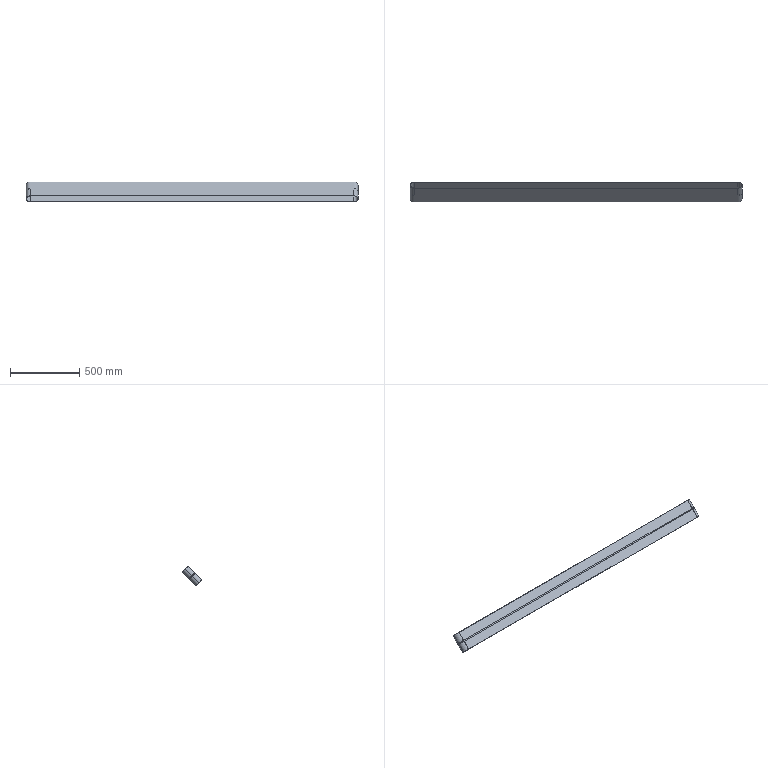Component | SolidWorks | Belt-2 | 1 solid | 32 faces | box 2398 x 143.9 x 143.9 mm | volume 1137609 mm3 | plane 14 | cylinder 12 | cone 6 | commonest cylinder face diameters 60 x6 52 x3 63 x3
build123d program:
from build123d import *

# Parameters (mm, degrees)
EXTRUDE_THIN1_DEPTH = 70


with BuildPart() as part:
    # Sketch1 → Extrude-Thin1 (new, symmetric)
    with BuildSketch(Plane.XY):
        with BuildLine():
            Line((-1167.5, 31.5), (1167.5, 31.5))
            ThreePointArc((1167.5, 31.5), (1199, 0), (1167.5, -31.5))
            Line((1167.5, -31.5), (-1167.5, -31.5))
            ThreePointArc((-1167.5, -31.5), (-1199, 0), (-1167.5, 31.5))
        make_face()
        with BuildLine():
            Line((-1167.5, 30), (1167.5, 30))
            ThreePointArc((1167.5, 30), (1197.5, 0), (1167.5, -30))
            Line((1167.5, -30), (-1167.5, -30))
            ThreePointArc((-1167.5, -30), (-1197.5, 0), (-1167.5, 30))
        make_face(mode=Mode.SUBTRACT)
    extrude(amount=EXTRUDE_THIN1_DEPTH, both=True)

    # Sweep1: sweep along a path in Sketch3
    with BuildLine(Plane.XY) as sweep1_path:
        Line((-1167.5, 30), (1167.5, 30))
        ThreePointArc((1167.5, 30), (1197.5, 0), (1167.5, -30))
        Line((1167.5, -30), (-1167.5, -30))
        ThreePointArc((-1167.5, -30), (-1197.5, 0), (-1167.5, 30))
    # Sketch2 → Sweep1 (sweep)
    with BuildSketch(Plane(origin=(0, 0, 0), x_dir=(0, 0, -1), z_dir=(1, 0, 0))):
        Polygon((-4, -30), (4, -30), (2, -26), (-2, -26), align=None)
    sweep(path=sweep1_path.line)


solid = part.part

# Placed as in the assembly
solid = solid.moved(Location((1065.5, 709.045, 342.308), (-45, 0, -0.01232)))
STEP:
#1=CARTESIAN_POINT('',(-5.039,27.867,13.414));
#2=VERTEX_POINT('',#1);
#3=CARTESIAN_POINT('',(-4.016,28.59,12.69));
#4=VERTEX_POINT('',#3);
#5=CARTESIAN_POINT('',(-4.016,27.866,13.414));
#6=DIRECTION('',(0.,-0.7071,-0.7071));
#7=DIRECTION('',(-1.,0.000152,-0.000152));
#8=AXIS2_PLACEMENT_3D('',#5,#6,#7);
#9=CIRCLE('',#8,1.024);
#10=EDGE_CURVE('',#2,#4,#9,.T.);
#11=ORIENTED_EDGE('',*,*,#10,.F.);
#12=CARTESIAN_POINT('',(-5.197,27.811,13.358));
#13=VERTEX_POINT('',#12);
#14=CARTESIAN_POINT('',(-5.197,27.811,13.358));
#15=DIRECTION('',(-0.8944,-0.3161,-0.3164));
#16=VECTOR('',#15,39.37);
#17=LINE('',#14,#16);
#18=EDGE_CURVE('',#2,#13,#17,.T.);
#19=ORIENTED_EDGE('',*,*,#18,.T.);
#20=CARTESIAN_POINT('',(-4.015,28.646,12.523));
#21=VERTEX_POINT('',#20);
#22=CARTESIAN_POINT('',(-4.016,27.811,13.358));
#23=DIRECTION('',(0.,-0.7071,-0.7071));
#24=DIRECTION('',(-1.,0.000152,-0.000152));
#25=AXIS2_PLACEMENT_3D('',#22,#23,#24);
#26=CIRCLE('',#25,1.181);
#27=EDGE_CURVE('',#13,#21,#26,.T.);
#28=ORIENTED_EDGE('',*,*,#27,.T.);
#29=CARTESIAN_POINT('',(-4.015,28.646,12.523));
#30=DIRECTION('',(-0.0001923,-0.3162,0.9487));
#31=VECTOR('',#30,39.37);
#32=LINE('',#29,#31);
#33=EDGE_CURVE('',#21,#4,#32,.T.);
#34=ORIENTED_EDGE('',*,*,#33,.T.);
#35=EDGE_LOOP('',(#11,#19,#28,#34));
#36=FACE_OUTER_BOUND('',#35,.T.);
#37=CARTESIAN_POINT('',(-4.016,27.811,13.358));
#38=DIRECTION('',(0.,-0.7071,-0.7071));
#39=DIRECTION('',(-1.,0.000152,-0.000152));
#40=AXIS2_PLACEMENT_3D('',#37,#38,#39);
#41=CONICAL_SURFACE('',#40,1.181,1.107);
#42=ADVANCED_FACE('',(#36),#41,.F.);
#43=CARTESIAN_POINT('',(-5.039,27.978,13.525));
#44=VERTEX_POINT('',#43);
#45=CARTESIAN_POINT('',(-4.016,28.702,12.802));
#46=VERTEX_POINT('',#45);
#47=CARTESIAN_POINT('',(-4.016,27.978,13.525));
#48=DIRECTION('',(0.,-0.7071,-0.7071));
#49=DIRECTION('',(-1.,0.000152,-0.000152));
#50=AXIS2_PLACEMENT_3D('',#47,#48,#49);
#51=CIRCLE('',#50,1.024);
#52=EDGE_CURVE('',#44,#46,#51,.T.);
#53=ORIENTED_EDGE('',*,*,#52,.F.);
#54=CARTESIAN_POINT('',(-5.039,27.922,13.47));
#55=DIRECTION('',(0.,-0.7071,-0.7071));
#56=VECTOR('',#55,39.37);
#57=LINE('',#54,#56);
#58=EDGE_CURVE('',#44,#2,#57,.T.);
#59=ORIENTED_EDGE('',*,*,#58,.T.);
#60=ORIENTED_EDGE('',*,*,#10,.T.);
#61=CARTESIAN_POINT('',(-4.016,28.59,12.69));
#62=DIRECTION('',(-0.,0.7071,0.7071));
#63=VECTOR('',#62,39.37);
#64=LINE('',#61,#63);
#65=EDGE_CURVE('',#4,#46,#64,.T.);
#66=ORIENTED_EDGE('',*,*,#65,.T.);
#67=EDGE_LOOP('',(#53,#59,#60,#66));
#68=FACE_OUTER_BOUND('',#67,.T.);
#69=CARTESIAN_POINT('',(-4.016,27.922,13.47));
#70=DIRECTION('',(0.,-0.7071,-0.7071));
#71=DIRECTION('',(-1.,0.000152,-0.000152));
#72=AXIS2_PLACEMENT_3D('',#69,#70,#71);
#73=CYLINDRICAL_SURFACE('',#72,1.024);
#74=ADVANCED_FACE('',(#68),#73,.F.);
#75=CARTESIAN_POINT('',(87.914,28.688,12.816));
#76=VERTEX_POINT('',#75);
#77=CARTESIAN_POINT('',(88.937,27.964,13.54));
#78=VERTEX_POINT('',#77);
#79=CARTESIAN_POINT('',(87.913,27.964,13.539));
#80=DIRECTION('',(0.,-0.7071,-0.7071));
#81=DIRECTION('',(-1.,0.000152,-0.000152));
#82=AXIS2_PLACEMENT_3D('',#79,#80,#81);
#83=CIRCLE('',#82,1.024);
#84=EDGE_CURVE('',#76,#78,#83,.T.);
#85=ORIENTED_EDGE('',*,*,#84,.T.);
#86=CARTESIAN_POINT('',(89.094,28.019,13.595));
#87=VERTEX_POINT('',#86);
#88=CARTESIAN_POINT('',(88.937,27.964,13.54));
#89=DIRECTION('',(0.8944,0.3161,0.3164));
#90=VECTOR('',#89,39.37);
#91=LINE('',#88,#90);
#92=EDGE_CURVE('',#78,#87,#91,.T.);
#93=ORIENTED_EDGE('',*,*,#92,.T.);
#94=CARTESIAN_POINT('',(87.914,28.855,12.76));
#95=VERTEX_POINT('',#94);
#96=CARTESIAN_POINT('',(87.913,28.02,13.595));
#97=DIRECTION('',(0.,-0.7071,-0.7071));
#98=DIRECTION('',(-1.,0.000152,-0.000152));
#99=AXIS2_PLACEMENT_3D('',#96,#97,#98);
#100=CIRCLE('',#99,1.181);
#101=EDGE_CURVE('',#95,#87,#100,.T.);
#102=ORIENTED_EDGE('',*,*,#101,.F.);
#103=CARTESIAN_POINT('',(87.914,28.688,12.816));
#104=DIRECTION('',(0.0001923,0.9487,-0.3162));
#105=VECTOR('',#104,39.37);
#106=LINE('',#103,#105);
#107=EDGE_CURVE('',#76,#95,#106,.T.);
#108=ORIENTED_EDGE('',*,*,#107,.F.);
#109=EDGE_LOOP('',(#85,#93,#102,#108));
#110=FACE_OUTER_BOUND('',#109,.T.);
#111=CARTESIAN_POINT('',(87.913,27.964,13.539));
#112=DIRECTION('',(-0.,0.7071,0.7071));
#113=DIRECTION('',(1.,-0.000152,0.000152));
#114=AXIS2_PLACEMENT_3D('',#111,#112,#113);
#115=CONICAL_SURFACE('',#114,1.024,1.107);
#116=ADVANCED_FACE('',(#110),#115,.F.);
#117=CARTESIAN_POINT('',(-5.256,29.871,15.418));
#118=VERTEX_POINT('',#117);
#119=CARTESIAN_POINT('',(-4.016,28.994,16.295));
#120=VERTEX_POINT('',#119);
#121=CARTESIAN_POINT('',(-4.016,29.871,15.418));
#122=DIRECTION('',(-0.,0.7071,0.7071));
#123=DIRECTION('',(1.,-0.000152,0.000152));
#124=AXIS2_PLACEMENT_3D('',#121,#122,#123);
#125=CIRCLE('',#124,1.24);
#126=EDGE_CURVE('',#118,#120,#125,.T.);
#127=ORIENTED_EDGE('',*,*,#126,.F.);
#128=CARTESIAN_POINT('',(-5.256,25.974,11.521));
#129=VERTEX_POINT('',#128);
#130=CARTESIAN_POINT('',(-5.256,29.871,15.418));
#131=DIRECTION('',(0.,-0.7071,-0.7071));
#132=VECTOR('',#131,39.37);
#133=LINE('',#130,#132);
#134=EDGE_CURVE('',#118,#129,#133,.T.);
#135=ORIENTED_EDGE('',*,*,#134,.T.);
#136=CARTESIAN_POINT('',(-4.016,25.096,12.398));
#137=VERTEX_POINT('',#136);
#138=CARTESIAN_POINT('',(-4.016,25.973,11.521));
#139=DIRECTION('',(-0.,0.7071,0.7071));
#140=DIRECTION('',(1.,-0.000152,0.000152));
#141=AXIS2_PLACEMENT_3D('',#138,#139,#140);
#142=CIRCLE('',#141,1.24);
#143=EDGE_CURVE('',#129,#137,#142,.T.);
#144=ORIENTED_EDGE('',*,*,#143,.T.);
#145=CARTESIAN_POINT('',(-4.016,28.994,16.295));
#146=DIRECTION('',(0.,-0.7071,-0.7071));
#147=VECTOR('',#146,39.37);
#148=LINE('',#145,#147);
#149=EDGE_CURVE('',#120,#137,#148,.T.);
#150=ORIENTED_EDGE('',*,*,#149,.F.);
#151=EDGE_LOOP('',(#127,#135,#144,#150));
#152=FACE_OUTER_BOUND('',#151,.T.);
#153=CARTESIAN_POINT('',(-4.016,29.871,15.418));
#154=DIRECTION('',(0.,-0.7071,-0.7071));
#155=DIRECTION('',(-1.,0.000152,-0.000152));
#156=AXIS2_PLACEMENT_3D('',#153,#154,#155);
#157=CYLINDRICAL_SURFACE('',#156,1.24);
#158=ADVANCED_FACE('',(#152),#157,.T.);
#159=CARTESIAN_POINT('',(-4.015,30.706,14.583));
#160=VERTEX_POINT('',#159);
#161=CARTESIAN_POINT('',(-5.197,29.871,15.418));
#162=VERTEX_POINT('',#161);
#163=CARTESIAN_POINT('',(-4.016,29.871,15.418));
#164=DIRECTION('',(-0.,0.7071,0.7071));
#165=DIRECTION('',(1.,-0.000152,0.000152));
#166=AXIS2_PLACEMENT_3D('',#163,#164,#165);
#167=CIRCLE('',#166,1.181);
#168=EDGE_CURVE('',#160,#162,#167,.T.);
#169=ORIENTED_EDGE('',*,*,#168,.T.);
#170=CARTESIAN_POINT('',(-5.197,28.034,13.581));
#171=VERTEX_POINT('',#170);
#172=CARTESIAN_POINT('',(-5.197,29.871,15.418));
#173=DIRECTION('',(0.,-0.7071,-0.7071));
#174=VECTOR('',#173,39.37);
#175=LINE('',#172,#174);
#176=EDGE_CURVE('',#162,#171,#175,.T.);
#177=ORIENTED_EDGE('',*,*,#176,.T.);
#178=CARTESIAN_POINT('',(-4.015,28.869,12.746));
#179=VERTEX_POINT('',#178);
#180=CARTESIAN_POINT('',(-4.016,28.033,13.581));
#181=DIRECTION('',(0.,-0.7071,-0.7071));
#182=DIRECTION('',(-1.,0.000152,-0.000152));
#183=AXIS2_PLACEMENT_3D('',#180,#181,#182);
#184=CIRCLE('',#183,1.181);
#185=EDGE_CURVE('',#171,#179,#184,.T.);
#186=ORIENTED_EDGE('',*,*,#185,.T.);
#187=CARTESIAN_POINT('',(-4.015,30.706,14.583));
#188=DIRECTION('',(0.,-0.7071,-0.7071));
#189=VECTOR('',#188,39.37);
#190=LINE('',#187,#189);
#191=EDGE_CURVE('',#160,#179,#190,.T.);
#192=ORIENTED_EDGE('',*,*,#191,.F.);
#193=EDGE_LOOP('',(#169,#177,#186,#192));
#194=FACE_OUTER_BOUND('',#193,.T.);
#195=CARTESIAN_POINT('',(-4.016,29.871,15.418));
#196=DIRECTION('',(0.,-0.7071,-0.7071));
#197=DIRECTION('',(-1.,0.000152,-0.000152));
#198=AXIS2_PLACEMENT_3D('',#195,#196,#197);
#199=CYLINDRICAL_SURFACE('',#198,1.181);
#200=ADVANCED_FACE('',(#194),#199,.F.);
#201=ORIENTED_EDGE('',*,*,#27,.F.);
#202=CARTESIAN_POINT('',(-5.197,25.974,11.521));
#203=VERTEX_POINT('',#202);
#204=CARTESIAN_POINT('',(-5.197,29.871,15.418));
#205=DIRECTION('',(0.,-0.7071,-0.7071));
#206=VECTOR('',#205,39.37);
#207=LINE('',#204,#206);
#208=EDGE_CURVE('',#13,#203,#207,.T.);
#209=ORIENTED_EDGE('',*,*,#208,.T.);
#210=CARTESIAN_POINT('',(-4.015,26.809,10.686));
#211=VERTEX_POINT('',#210);
#212=CARTESIAN_POINT('',(-4.016,25.973,11.521));
#213=DIRECTION('',(-0.,0.7071,0.7071));
#214=DIRECTION('',(1.,-0.000152,0.000152));
#215=AXIS2_PLACEMENT_3D('',#212,#213,#214);
#216=CIRCLE('',#215,1.181);
#217=EDGE_CURVE('',#211,#203,#216,.T.);
#218=ORIENTED_EDGE('',*,*,#217,.F.);
#219=CARTESIAN_POINT('',(-4.015,30.706,14.583));
#220=DIRECTION('',(0.,-0.7071,-0.7071));
#221=VECTOR('',#220,39.37);
#222=LINE('',#219,#221);
#223=EDGE_CURVE('',#21,#211,#222,.T.);
#224=ORIENTED_EDGE('',*,*,#223,.F.);
#225=EDGE_LOOP('',(#201,#209,#218,#224));
#226=FACE_OUTER_BOUND('',#225,.T.);
#227=CARTESIAN_POINT('',(-4.016,29.871,15.418));
#228=DIRECTION('',(0.,-0.7071,-0.7071));
#229=DIRECTION('',(-1.,0.000152,-0.000152));
#230=AXIS2_PLACEMENT_3D('',#227,#228,#229);
#231=CYLINDRICAL_SURFACE('',#230,1.181);
#232=ADVANCED_FACE('',(#226),#231,.F.);
#233=ORIENTED_EDGE('',*,*,#208,.F.);
#234=CARTESIAN_POINT('',(-4.016,26.976,14.194));
#235=VERTEX_POINT('',#234);
#236=CARTESIAN_POINT('',(-4.016,27.811,13.358));
#237=DIRECTION('',(0.,-0.7071,-0.7071));
#238=DIRECTION('',(-1.,0.000152,-0.000152));
#239=AXIS2_PLACEMENT_3D('',#236,#237,#238);
#240=CIRCLE('',#239,1.181);
#241=EDGE_CURVE('',#235,#13,#240,.T.);
#242=ORIENTED_EDGE('',*,*,#241,.F.);
#243=CARTESIAN_POINT('',(-4.016,25.138,12.356));
#244=VERTEX_POINT('',#243);
#245=CARTESIAN_POINT('',(-4.016,29.036,16.254));
#246=DIRECTION('',(0.,-0.7071,-0.7071));
#247=VECTOR('',#246,39.37);
#248=LINE('',#245,#247);
#249=EDGE_CURVE('',#235,#244,#248,.T.);
#250=ORIENTED_EDGE('',*,*,#249,.T.);
#251=CARTESIAN_POINT('',(-4.016,25.973,11.521));
#252=DIRECTION('',(-0.,0.7071,0.7071));
#253=DIRECTION('',(1.,-0.000152,0.000152));
#254=AXIS2_PLACEMENT_3D('',#251,#252,#253);
#255=CIRCLE('',#254,1.181);
#256=EDGE_CURVE('',#203,#244,#255,.T.);
#257=ORIENTED_EDGE('',*,*,#256,.F.);
#258=EDGE_LOOP('',(#233,#242,#250,#257));
#259=FACE_OUTER_BOUND('',#258,.T.);
#260=CARTESIAN_POINT('',(-4.016,29.871,15.418));
#261=DIRECTION('',(0.,-0.7071,-0.7071));
#262=DIRECTION('',(-1.,0.000152,-0.000152));
#263=AXIS2_PLACEMENT_3D('',#260,#261,#262);
#264=CYLINDRICAL_SURFACE('',#263,1.181);
#265=ADVANCED_FACE('',(#259),#264,.F.);
#266=ORIENTED_EDGE('',*,*,#176,.F.);
#267=CARTESIAN_POINT('',(-4.016,29.036,16.254));
#268=VERTEX_POINT('',#267);
#269=CARTESIAN_POINT('',(-4.016,29.871,15.418));
#270=DIRECTION('',(-0.,0.7071,0.7071));
#271=DIRECTION('',(1.,-0.000152,0.000152));
#272=AXIS2_PLACEMENT_3D('',#269,#270,#271);
#273=CIRCLE('',#272,1.181);
#274=EDGE_CURVE('',#162,#268,#273,.T.);
#275=ORIENTED_EDGE('',*,*,#274,.T.);
#276=CARTESIAN_POINT('',(-4.016,27.198,14.416));
#277=VERTEX_POINT('',#276);
#278=CARTESIAN_POINT('',(-4.016,29.036,16.254));
#279=DIRECTION('',(0.,-0.7071,-0.7071));
#280=VECTOR('',#279,39.37);
#281=LINE('',#278,#280);
#282=EDGE_CURVE('',#268,#277,#281,.T.);
#283=ORIENTED_EDGE('',*,*,#282,.T.);
#284=CARTESIAN_POINT('',(-4.016,28.033,13.581));
#285=DIRECTION('',(0.,-0.7071,-0.7071));
#286=DIRECTION('',(-1.,0.000152,-0.000152));
#287=AXIS2_PLACEMENT_3D('',#284,#285,#286);
#288=CIRCLE('',#287,1.181);
#289=EDGE_CURVE('',#277,#171,#288,.T.);
#290=ORIENTED_EDGE('',*,*,#289,.T.);
#291=EDGE_LOOP('',(#266,#275,#283,#290));
#292=FACE_OUTER_BOUND('',#291,.T.);
#293=CARTESIAN_POINT('',(-4.016,29.871,15.418));
#294=DIRECTION('',(0.,-0.7071,-0.7071));
#295=DIRECTION('',(-1.,0.000152,-0.000152));
#296=AXIS2_PLACEMENT_3D('',#293,#294,#295);
#297=CYLINDRICAL_SURFACE('',#296,1.181);
#298=ADVANCED_FACE('',(#292),#297,.F.);
#299=CARTESIAN_POINT('',(87.913,27.184,14.43));
#300=VERTEX_POINT('',#299);
#301=CARTESIAN_POINT('',(-4.016,27.198,14.416));
#302=DIRECTION('',(1.,-0.000152,0.000152));
#303=VECTOR('',#302,39.37);
#304=LINE('',#301,#303);
#305=EDGE_CURVE('',#277,#300,#304,.T.);
#306=ORIENTED_EDGE('',*,*,#305,.F.);
#307=ORIENTED_EDGE('',*,*,#282,.F.);
#308=CARTESIAN_POINT('',(87.913,29.022,16.268));
#309=VERTEX_POINT('',#308);
#310=CARTESIAN_POINT('',(87.913,29.022,16.268));
#311=DIRECTION('',(1.,-0.000152,0.000152));
#312=VECTOR('',#311,39.37);
#313=LINE('',#310,#312);
#314=EDGE_CURVE('',#268,#309,#313,.T.);
#315=ORIENTED_EDGE('',*,*,#314,.T.);
#316=CARTESIAN_POINT('',(87.913,29.022,16.268));
#317=DIRECTION('',(0.,-0.7071,-0.7071));
#318=VECTOR('',#317,39.37);
#319=LINE('',#316,#318);
#320=EDGE_CURVE('',#309,#300,#319,.T.);
#321=ORIENTED_EDGE('',*,*,#320,.T.);
#322=EDGE_LOOP('',(#306,#307,#315,#321));
#323=FACE_OUTER_BOUND('',#322,.T.);
#324=CARTESIAN_POINT('',(87.913,29.022,16.268));
#325=DIRECTION('',(0.000215,0.7071,-0.7071));
#326=DIRECTION('',(-0.,0.7071,0.7071));
#327=AXIS2_PLACEMENT_3D('',#324,#325,#326);
#328=PLANE('',#327);
#329=ADVANCED_FACE('',(#323),#328,.T.);
#330=CARTESIAN_POINT('',(87.913,26.962,14.207));
#331=VERTEX_POINT('',#330);
#332=CARTESIAN_POINT('',(87.913,25.124,12.37));
#333=VERTEX_POINT('',#332);
#334=CARTESIAN_POINT('',(87.913,29.022,16.268));
#335=DIRECTION('',(0.,-0.7071,-0.7071));
#336=VECTOR('',#335,39.37);
#337=LINE('',#334,#336);
#338=EDGE_CURVE('',#331,#333,#337,.T.);
#339=ORIENTED_EDGE('',*,*,#338,.F.);
#340=CARTESIAN_POINT('',(87.914,28.632,12.537));
#341=VERTEX_POINT('',#340);
#342=CARTESIAN_POINT('',(87.913,27.797,13.372));
#343=DIRECTION('',(0.,-0.7071,-0.7071));
#344=DIRECTION('',(-1.,0.000152,-0.000152));
#345=AXIS2_PLACEMENT_3D('',#342,#343,#344);
#346=CIRCLE('',#345,1.181);
#347=EDGE_CURVE('',#341,#331,#346,.T.);
#348=ORIENTED_EDGE('',*,*,#347,.F.);
#349=CARTESIAN_POINT('',(87.914,26.795,10.7));
#350=VERTEX_POINT('',#349);
#351=CARTESIAN_POINT('',(87.914,30.692,14.597));
#352=DIRECTION('',(0.,-0.7071,-0.7071));
#353=VECTOR('',#352,39.37);
#354=LINE('',#351,#353);
#355=EDGE_CURVE('',#341,#350,#354,.T.);
#356=ORIENTED_EDGE('',*,*,#355,.T.);
#357=CARTESIAN_POINT('',(87.913,25.959,11.535));
#358=DIRECTION('',(-0.,0.7071,0.7071));
#359=DIRECTION('',(1.,-0.000152,0.000152));
#360=AXIS2_PLACEMENT_3D('',#357,#358,#359);
#361=CIRCLE('',#360,1.181);
#362=EDGE_CURVE('',#333,#350,#361,.T.);
#363=ORIENTED_EDGE('',*,*,#362,.F.);
#364=EDGE_LOOP('',(#339,#348,#356,#363));
#365=FACE_OUTER_BOUND('',#364,.T.);
#366=CARTESIAN_POINT('',(87.913,29.857,15.432));
#367=DIRECTION('',(0.,-0.7071,-0.7071));
#368=DIRECTION('',(-1.,0.000152,-0.000152));
#369=AXIS2_PLACEMENT_3D('',#366,#367,#368);
#370=CYLINDRICAL_SURFACE('',#369,1.181);
#371=ADVANCED_FACE('',(#365),#370,.F.);
#372=CARTESIAN_POINT('',(87.914,30.692,14.597));
#373=VERTEX_POINT('',#372);
#374=CARTESIAN_POINT('',(87.914,30.692,14.597));
#375=DIRECTION('',(0.,-0.7071,-0.7071));
#376=VECTOR('',#375,39.37);
#377=LINE('',#374,#376);
#378=EDGE_CURVE('',#373,#95,#377,.T.);
#379=ORIENTED_EDGE('',*,*,#378,.T.);
#380=ORIENTED_EDGE('',*,*,#101,.T.);
#381=CARTESIAN_POINT('',(87.913,28.02,13.595));
#382=DIRECTION('',(0.,-0.7071,-0.7071));
#383=DIRECTION('',(-1.,0.000152,-0.000152));
#384=AXIS2_PLACEMENT_3D('',#381,#382,#383);
#385=CIRCLE('',#384,1.181);
#386=EDGE_CURVE('',#87,#300,#385,.T.);
#387=ORIENTED_EDGE('',*,*,#386,.T.);
#388=ORIENTED_EDGE('',*,*,#320,.F.);
#389=CARTESIAN_POINT('',(87.913,29.857,15.432));
#390=DIRECTION('',(-0.,0.7071,0.7071));
#391=DIRECTION('',(1.,-0.000152,0.000152));
#392=AXIS2_PLACEMENT_3D('',#389,#390,#391);
#393=CIRCLE('',#392,1.181);
#394=EDGE_CURVE('',#309,#373,#393,.T.);
#395=ORIENTED_EDGE('',*,*,#394,.T.);
#396=EDGE_LOOP('',(#379,#380,#387,#388,#395));
#397=FACE_OUTER_BOUND('',#396,.T.);
#398=CARTESIAN_POINT('',(87.913,29.857,15.432));
#399=DIRECTION('',(0.,-0.7071,-0.7071));
#400=DIRECTION('',(-1.,0.000152,-0.000152));
#401=AXIS2_PLACEMENT_3D('',#398,#399,#400);
#402=CYLINDRICAL_SURFACE('',#401,1.181);
#403=ADVANCED_FACE('',(#397),#402,.F.);
#404=ORIENTED_EDGE('',*,*,#355,.F.);
#405=CARTESIAN_POINT('',(-4.015,28.646,12.523));
#406=DIRECTION('',(1.,-0.000152,0.000152));
#407=VECTOR('',#406,39.37);
#408=LINE('',#405,#407);
#409=EDGE_CURVE('',#21,#341,#408,.T.);
#410=ORIENTED_EDGE('',*,*,#409,.F.);
#411=ORIENTED_EDGE('',*,*,#223,.T.);
#412=CARTESIAN_POINT('',(-4.015,26.809,10.686));
#413=DIRECTION('',(-1.,0.000152,-0.000152));
#414=VECTOR('',#413,39.37);
#415=LINE('',#412,#414);
#416=EDGE_CURVE('',#350,#211,#415,.T.);
#417=ORIENTED_EDGE('',*,*,#416,.F.);
#418=EDGE_LOOP('',(#404,#410,#411,#417));
#419=FACE_OUTER_BOUND('',#418,.T.);
#420=CARTESIAN_POINT('',(-4.015,30.706,14.583));
#421=DIRECTION('',(-0.000215,-0.7071,0.7071));
#422=DIRECTION('',(0.,-0.7071,-0.7071));
#423=AXIS2_PLACEMENT_3D('',#420,#421,#422);
#424=PLANE('',#423);
#425=ADVANCED_FACE('',(#419),#424,.T.);
#426=ORIENTED_EDGE('',*,*,#191,.T.);
#427=CARTESIAN_POINT('',(-4.015,28.869,12.746));
#428=DIRECTION('',(1.,-0.000152,0.000152));
#429=VECTOR('',#428,39.37);
#430=LINE('',#427,#429);
#431=EDGE_CURVE('',#179,#95,#430,.T.);
#432=ORIENTED_EDGE('',*,*,#431,.T.);
#433=ORIENTED_EDGE('',*,*,#378,.F.);
#434=CARTESIAN_POINT('',(-4.015,30.706,14.583));
#435=DIRECTION('',(-1.,0.000152,-0.000152));
#436=VECTOR('',#435,39.37);
#437=LINE('',#434,#436);
#438=EDGE_CURVE('',#373,#160,#437,.T.);
#439=ORIENTED_EDGE('',*,*,#438,.T.);
#440=EDGE_LOOP('',(#426,#432,#433,#439));
#441=FACE_OUTER_BOUND('',#440,.T.);
#442=CARTESIAN_POINT('',(-4.015,30.706,14.583));
#443=DIRECTION('',(-0.000215,-0.7071,0.7071));
#444=DIRECTION('',(0.,-0.7071,-0.7071));
#445=AXIS2_PLACEMENT_3D('',#442,#443,#444);
#446=PLANE('',#445);
#447=ADVANCED_FACE('',(#441),#446,.T.);
#448=CARTESIAN_POINT('',(-4.015,30.748,14.541));
#449=VERTEX_POINT('',#448);
#450=CARTESIAN_POINT('',(-4.016,29.871,15.418));
#451=DIRECTION('',(-0.,0.7071,0.7071));
#452=DIRECTION('',(1.,-0.000152,0.000152));
#453=AXIS2_PLACEMENT_3D('',#450,#451,#452);
#454=CIRCLE('',#453,1.24);
#455=EDGE_CURVE('',#449,#118,#454,.T.);
#456=ORIENTED_EDGE('',*,*,#455,.T.);
#457=ORIENTED_EDGE('',*,*,#126,.T.);
#458=CARTESIAN_POINT('',(87.913,28.98,16.309));
#459=VERTEX_POINT('',#458);
#460=CARTESIAN_POINT('',(87.913,28.98,16.309));
#461=DIRECTION('',(1.,-0.000152,0.000152));
#462=VECTOR('',#461,39.37);
#463=LINE('',#460,#462);
#464=EDGE_CURVE('',#120,#459,#463,.T.);
#465=ORIENTED_EDGE('',*,*,#464,.T.);
#466=CARTESIAN_POINT('',(87.914,30.734,14.555));
#467=VERTEX_POINT('',#466);
#468=CARTESIAN_POINT('',(87.913,29.857,15.432));
#469=DIRECTION('',(-0.,0.7071,0.7071));
#470=DIRECTION('',(1.,-0.000152,0.000152));
#471=AXIS2_PLACEMENT_3D('',#468,#469,#470);
#472=CIRCLE('',#471,1.24);
#473=EDGE_CURVE('',#459,#467,#472,.T.);
#474=ORIENTED_EDGE('',*,*,#473,.T.);
#475=CARTESIAN_POINT('',(-4.015,30.748,14.541));
#476=DIRECTION('',(-1.,0.000152,-0.000152));
#477=VECTOR('',#476,39.37);
#478=LINE('',#475,#477);
#479=EDGE_CURVE('',#467,#449,#478,.T.);
#480=ORIENTED_EDGE('',*,*,#479,.T.);
#481=EDGE_LOOP('',(#456,#457,#465,#474,#480));
#482=FACE_OUTER_BOUND('',#481,.T.);
#483=ORIENTED_EDGE('',*,*,#314,.F.);
#484=ORIENTED_EDGE('',*,*,#274,.F.);
#485=ORIENTED_EDGE('',*,*,#168,.F.);
#486=ORIENTED_EDGE('',*,*,#438,.F.);
#487=ORIENTED_EDGE('',*,*,#394,.F.);
#488=EDGE_LOOP('',(#483,#484,#485,#486,#487));
#489=FACE_BOUND('',#488,.T.);
#490=CARTESIAN_POINT('',(-4.016,29.871,15.418));
#491=DIRECTION('',(-0.,0.7071,0.7071));
#492=DIRECTION('',(1.,-0.000152,0.000152));
#493=AXIS2_PLACEMENT_3D('',#490,#491,#492);
#494=PLANE('',#493);
#495=ADVANCED_FACE('',(#482,#489),#494,.T.);
#496=CARTESIAN_POINT('',(-4.015,26.85,10.644));
#497=VERTEX_POINT('',#496);
#498=CARTESIAN_POINT('',(-4.016,25.973,11.521));
#499=DIRECTION('',(-0.,0.7071,0.7071));
#500=DIRECTION('',(1.,-0.000152,0.000152));
#501=AXIS2_PLACEMENT_3D('',#498,#499,#500);
#502=CIRCLE('',#501,1.24);
#503=EDGE_CURVE('',#497,#129,#502,.T.);
#504=ORIENTED_EDGE('',*,*,#503,.F.);
#505=CARTESIAN_POINT('',(87.914,26.836,10.658));
#506=VERTEX_POINT('',#505);
#507=CARTESIAN_POINT('',(-4.015,26.85,10.644));
#508=DIRECTION('',(-1.,0.000152,-0.000152));
#509=VECTOR('',#508,39.37);
#510=LINE('',#507,#509);
#511=EDGE_CURVE('',#506,#497,#510,.T.);
#512=ORIENTED_EDGE('',*,*,#511,.F.);
#513=CARTESIAN_POINT('',(87.913,25.083,12.412));
#514=VERTEX_POINT('',#513);
#515=CARTESIAN_POINT('',(87.913,25.959,11.535));
#516=DIRECTION('',(-0.,0.7071,0.7071));
#517=DIRECTION('',(1.,-0.000152,0.000152));
#518=AXIS2_PLACEMENT_3D('',#515,#516,#517);
#519=CIRCLE('',#518,1.24);
#520=EDGE_CURVE('',#514,#506,#519,.T.);
#521=ORIENTED_EDGE('',*,*,#520,.F.);
#522=CARTESIAN_POINT('',(87.913,25.083,12.412));
#523=DIRECTION('',(1.,-0.000152,0.000152));
#524=VECTOR('',#523,39.37);
#525=LINE('',#522,#524);
#526=EDGE_CURVE('',#137,#514,#525,.T.);
#527=ORIENTED_EDGE('',*,*,#526,.F.);
#528=ORIENTED_EDGE('',*,*,#143,.F.);
#529=EDGE_LOOP('',(#504,#512,#521,#527,#528));
#530=FACE_OUTER_BOUND('',#529,.T.);
#531=ORIENTED_EDGE('',*,*,#217,.T.);
#532=ORIENTED_EDGE('',*,*,#256,.T.);
#533=CARTESIAN_POINT('',(87.913,25.124,12.37));
#534=DIRECTION('',(1.,-0.000152,0.000152));
#535=VECTOR('',#534,39.37);
#536=LINE('',#533,#535);
#537=EDGE_CURVE('',#244,#333,#536,.T.);
#538=ORIENTED_EDGE('',*,*,#537,.T.);
#539=ORIENTED_EDGE('',*,*,#362,.T.);
#540=ORIENTED_EDGE('',*,*,#416,.T.);
#541=EDGE_LOOP('',(#531,#532,#538,#539,#540));
#542=FACE_BOUND('',#541,.T.);
#543=CARTESIAN_POINT('',(-4.016,25.973,11.521));
#544=DIRECTION('',(-0.,0.7071,0.7071));
#545=DIRECTION('',(1.,-0.000152,0.000152));
#546=AXIS2_PLACEMENT_3D('',#543,#544,#545);
#547=PLANE('',#546);
#548=ADVANCED_FACE('',(#530,#542),#547,.F.);
#549=ORIENTED_EDGE('',*,*,#134,.F.);
#550=ORIENTED_EDGE('',*,*,#455,.F.);
#551=CARTESIAN_POINT('',(-4.015,30.748,14.541));
#552=DIRECTION('',(0.,-0.7071,-0.7071));
#553=VECTOR('',#552,39.37);
#554=LINE('',#551,#553);
#555=EDGE_CURVE('',#449,#497,#554,.T.);
#556=ORIENTED_EDGE('',*,*,#555,.T.);
#557=ORIENTED_EDGE('',*,*,#503,.T.);
#558=EDGE_LOOP('',(#549,#550,#556,#557));
#559=FACE_OUTER_BOUND('',#558,.T.);
#560=CARTESIAN_POINT('',(-4.016,29.871,15.418));
#561=DIRECTION('',(0.,-0.7071,-0.7071));
#562=DIRECTION('',(-1.,0.000152,-0.000152));
#563=AXIS2_PLACEMENT_3D('',#560,#561,#562);
#564=CYLINDRICAL_SURFACE('',#563,1.24);
#565=ADVANCED_FACE('',(#559),#564,.T.);
#566=ORIENTED_EDGE('',*,*,#526,.T.);
#567=CARTESIAN_POINT('',(87.913,28.98,16.309));
#568=DIRECTION('',(0.,-0.7071,-0.7071));
#569=VECTOR('',#568,39.37);
#570=LINE('',#567,#569);
#571=EDGE_CURVE('',#459,#514,#570,.T.);
#572=ORIENTED_EDGE('',*,*,#571,.F.);
#573=ORIENTED_EDGE('',*,*,#464,.F.);
#574=ORIENTED_EDGE('',*,*,#149,.T.);
#575=EDGE_LOOP('',(#566,#572,#573,#574));
#576=FACE_OUTER_BOUND('',#575,.T.);
#577=CARTESIAN_POINT('',(87.913,28.98,16.309));
#578=DIRECTION('',(0.000215,0.7071,-0.7071));
#579=DIRECTION('',(-0.,0.7071,0.7071));
#580=AXIS2_PLACEMENT_3D('',#577,#578,#579);
#581=PLANE('',#580);
#582=ADVANCED_FACE('',(#576),#581,.F.);
#583=ORIENTED_EDGE('',*,*,#520,.T.);
#584=CARTESIAN_POINT('',(87.914,30.734,14.555));
#585=DIRECTION('',(0.,-0.7071,-0.7071));
#586=VECTOR('',#585,39.37);
#587=LINE('',#584,#586);
#588=EDGE_CURVE('',#467,#506,#587,.T.);
#589=ORIENTED_EDGE('',*,*,#588,.F.);
#590=ORIENTED_EDGE('',*,*,#473,.F.);
#591=ORIENTED_EDGE('',*,*,#571,.T.);
#592=EDGE_LOOP('',(#583,#589,#590,#591));
#593=FACE_OUTER_BOUND('',#592,.T.);
#594=CARTESIAN_POINT('',(87.913,29.857,15.432));
#595=DIRECTION('',(0.,-0.7071,-0.7071));
#596=DIRECTION('',(-1.,0.000152,-0.000152));
#597=AXIS2_PLACEMENT_3D('',#594,#595,#596);
#598=CYLINDRICAL_SURFACE('',#597,1.24);
#599=ADVANCED_FACE('',(#593),#598,.T.);
#600=ORIENTED_EDGE('',*,*,#511,.T.);
#601=ORIENTED_EDGE('',*,*,#555,.F.);
#602=ORIENTED_EDGE('',*,*,#479,.F.);
#603=ORIENTED_EDGE('',*,*,#588,.T.);
#604=EDGE_LOOP('',(#600,#601,#602,#603));
#605=FACE_OUTER_BOUND('',#604,.T.);
#606=CARTESIAN_POINT('',(-4.015,30.748,14.541));
#607=DIRECTION('',(-0.000215,-0.7071,0.7071));
#608=DIRECTION('',(0.,-0.7071,-0.7071));
#609=AXIS2_PLACEMENT_3D('',#606,#607,#608);
#610=PLANE('',#609);
#611=ADVANCED_FACE('',(#605),#610,.F.);
#612=CARTESIAN_POINT('',(-4.016,26.976,14.194));
#613=DIRECTION('',(1.,-0.000152,0.000152));
#614=VECTOR('',#613,39.37);
#615=LINE('',#612,#614);
#616=EDGE_CURVE('',#235,#331,#615,.T.);
#617=ORIENTED_EDGE('',*,*,#616,.T.);
#618=ORIENTED_EDGE('',*,*,#338,.T.);
#619=ORIENTED_EDGE('',*,*,#537,.F.);
#620=ORIENTED_EDGE('',*,*,#249,.F.);
#621=EDGE_LOOP('',(#617,#618,#619,#620));
#622=FACE_OUTER_BOUND('',#621,.T.);
#623=CARTESIAN_POINT('',(87.913,29.022,16.268));
#624=DIRECTION('',(0.000215,0.7071,-0.7071));
#625=DIRECTION('',(-0.,0.7071,0.7071));
#626=AXIS2_PLACEMENT_3D('',#623,#624,#625);
#627=PLANE('',#626);
#628=ADVANCED_FACE('',(#622),#627,.T.);
#629=CARTESIAN_POINT('',(87.914,28.576,12.704));
#630=VERTEX_POINT('',#629);
#631=CARTESIAN_POINT('',(87.914,28.576,12.704));
#632=DIRECTION('',(-0.,0.7071,0.7071));
#633=VECTOR('',#632,39.37);
#634=LINE('',#631,#633);
#635=EDGE_CURVE('',#630,#76,#634,.T.);
#636=ORIENTED_EDGE('',*,*,#635,.F.);
#637=CARTESIAN_POINT('',(87.913,27.129,14.152));
#638=VERTEX_POINT('',#637);
#639=CARTESIAN_POINT('',(87.913,27.852,13.428));
#640=DIRECTION('',(0.,-0.7071,-0.7071));
#641=DIRECTION('',(-1.,0.000152,-0.000152));
#642=AXIS2_PLACEMENT_3D('',#639,#640,#641);
#643=CIRCLE('',#642,1.024);
#644=EDGE_CURVE('',#630,#638,#643,.T.);
#645=ORIENTED_EDGE('',*,*,#644,.T.);
#646=CARTESIAN_POINT('',(87.913,27.24,14.263));
#647=VERTEX_POINT('',#646);
#648=CARTESIAN_POINT('',(87.913,27.129,14.152));
#649=DIRECTION('',(-0.,0.7071,0.7071));
#650=VECTOR('',#649,39.37);
#651=LINE('',#648,#650);
#652=EDGE_CURVE('',#638,#647,#651,.T.);
#653=ORIENTED_EDGE('',*,*,#652,.T.);
#654=CARTESIAN_POINT('',(87.913,27.964,13.539));
#655=DIRECTION('',(0.,-0.7071,-0.7071));
#656=DIRECTION('',(-1.,0.000152,-0.000152));
#657=AXIS2_PLACEMENT_3D('',#654,#655,#656);
#658=CIRCLE('',#657,1.024);
#659=EDGE_CURVE('',#78,#647,#658,.T.);
#660=ORIENTED_EDGE('',*,*,#659,.F.);
#661=ORIENTED_EDGE('',*,*,#84,.F.);
#662=EDGE_LOOP('',(#636,#645,#653,#660,#661));
#663=FACE_OUTER_BOUND('',#662,.T.);
#664=CARTESIAN_POINT('',(87.913,27.908,13.484));
#665=DIRECTION('',(0.,-0.7071,-0.7071));
#666=DIRECTION('',(-1.,0.000152,-0.000152));
#667=AXIS2_PLACEMENT_3D('',#664,#665,#666);
#668=CYLINDRICAL_SURFACE('',#667,1.024);
#669=ADVANCED_FACE('',(#663),#668,.F.);
#670=CARTESIAN_POINT('',(87.914,28.632,12.537));
#671=DIRECTION('',(-0.0001923,-0.3162,0.9487));
#672=VECTOR('',#671,39.37);
#673=LINE('',#670,#672);
#674=EDGE_CURVE('',#341,#630,#673,.T.);
#675=ORIENTED_EDGE('',*,*,#674,.F.);
#676=ORIENTED_EDGE('',*,*,#347,.T.);
#677=CARTESIAN_POINT('',(87.913,26.962,14.207));
#678=DIRECTION('',(0.0001923,0.9487,-0.3162));
#679=VECTOR('',#678,39.37);
#680=LINE('',#677,#679);
#681=EDGE_CURVE('',#331,#638,#680,.T.);
#682=ORIENTED_EDGE('',*,*,#681,.T.);
#683=ORIENTED_EDGE('',*,*,#644,.F.);
#684=EDGE_LOOP('',(#675,#676,#682,#683));
#685=FACE_OUTER_BOUND('',#684,.T.);
#686=CARTESIAN_POINT('',(87.913,27.797,13.372));
#687=DIRECTION('',(0.,-0.7071,-0.7071));
#688=DIRECTION('',(-1.,0.000152,-0.000152));
#689=AXIS2_PLACEMENT_3D('',#686,#687,#688);
#690=CONICAL_SURFACE('',#689,1.181,1.107);
#691=ADVANCED_FACE('',(#685),#690,.F.);
#692=ORIENTED_EDGE('',*,*,#92,.F.);
#693=ORIENTED_EDGE('',*,*,#659,.T.);
#694=CARTESIAN_POINT('',(87.913,27.24,14.263));
#695=DIRECTION('',(-0.0001923,-0.3162,0.9487));
#696=VECTOR('',#695,39.37);
#697=LINE('',#694,#696);
#698=EDGE_CURVE('',#647,#300,#697,.T.);
#699=ORIENTED_EDGE('',*,*,#698,.T.);
#700=ORIENTED_EDGE('',*,*,#386,.F.);
#701=EDGE_LOOP('',(#692,#693,#699,#700));
#702=FACE_OUTER_BOUND('',#701,.T.);
#703=CARTESIAN_POINT('',(87.913,27.964,13.539));
#704=DIRECTION('',(-0.,0.7071,0.7071));
#705=DIRECTION('',(1.,-0.000152,0.000152));
#706=AXIS2_PLACEMENT_3D('',#703,#704,#705);
#707=CONICAL_SURFACE('',#706,1.024,1.107);
#708=ADVANCED_FACE('',(#702),#707,.F.);
#709=ORIENTED_EDGE('',*,*,#65,.F.);
#710=CARTESIAN_POINT('',(-4.016,28.59,12.69));
#711=DIRECTION('',(1.,-0.000152,0.000152));
#712=VECTOR('',#711,39.37);
#713=LINE('',#710,#712);
#714=EDGE_CURVE('',#4,#630,#713,.T.);
#715=ORIENTED_EDGE('',*,*,#714,.T.);
#716=ORIENTED_EDGE('',*,*,#635,.T.);
#717=CARTESIAN_POINT('',(-4.016,28.702,12.802));
#718=DIRECTION('',(1.,-0.000152,0.000152));
#719=VECTOR('',#718,39.37);
#720=LINE('',#717,#719);
#721=EDGE_CURVE('',#46,#76,#720,.T.);
#722=ORIENTED_EDGE('',*,*,#721,.F.);
#723=EDGE_LOOP('',(#709,#715,#716,#722));
#724=FACE_OUTER_BOUND('',#723,.T.);
#725=CARTESIAN_POINT('',(-4.016,28.59,12.69));
#726=DIRECTION('',(0.000215,0.7071,-0.7071));
#727=DIRECTION('',(-0.,0.7071,0.7071));
#728=AXIS2_PLACEMENT_3D('',#725,#726,#727);
#729=PLANE('',#728);
#730=ADVANCED_FACE('',(#724),#729,.F.);
#731=ORIENTED_EDGE('',*,*,#33,.F.);
#732=ORIENTED_EDGE('',*,*,#409,.T.);
#733=ORIENTED_EDGE('',*,*,#674,.T.);
#734=ORIENTED_EDGE('',*,*,#714,.F.);
#735=EDGE_LOOP('',(#731,#732,#733,#734));
#736=FACE_OUTER_BOUND('',#735,.T.);
#737=CARTESIAN_POINT('',(-4.015,28.646,12.523));
#738=DIRECTION('',(0.00009615,0.9487,0.3162));
#739=DIRECTION('',(-0.0001923,-0.3162,0.9487));
#740=AXIS2_PLACEMENT_3D('',#737,#738,#739);
#741=PLANE('',#740);
#742=ADVANCED_FACE('',(#736),#741,.F.);
#743=CARTESIAN_POINT('',(-4.016,28.702,12.802));
#744=DIRECTION('',(0.0001923,0.9487,-0.3162));
#745=VECTOR('',#744,39.37);
#746=LINE('',#743,#745);
#747=EDGE_CURVE('',#46,#179,#746,.T.);
#748=ORIENTED_EDGE('',*,*,#747,.F.);
#749=ORIENTED_EDGE('',*,*,#721,.T.);
#750=ORIENTED_EDGE('',*,*,#107,.T.);
#751=ORIENTED_EDGE('',*,*,#431,.F.);
#752=EDGE_LOOP('',(#748,#749,#750,#751));
#753=FACE_OUTER_BOUND('',#752,.T.);
#754=CARTESIAN_POINT('',(-4.016,28.702,12.802));
#755=DIRECTION('',(0.00009615,-0.3162,-0.9487));
#756=DIRECTION('',(0.0001923,0.9487,-0.3162));
#757=AXIS2_PLACEMENT_3D('',#754,#755,#756);
#758=PLANE('',#757);
#759=ADVANCED_FACE('',(#753),#758,.F.);
#760=ORIENTED_EDGE('',*,*,#58,.F.);
#761=CARTESIAN_POINT('',(-4.016,27.254,14.249));
#762=VERTEX_POINT('',#761);
#763=CARTESIAN_POINT('',(-4.016,27.978,13.525));
#764=DIRECTION('',(0.,-0.7071,-0.7071));
#765=DIRECTION('',(-1.,0.000152,-0.000152));
#766=AXIS2_PLACEMENT_3D('',#763,#764,#765);
#767=CIRCLE('',#766,1.024);
#768=EDGE_CURVE('',#762,#44,#767,.T.);
#769=ORIENTED_EDGE('',*,*,#768,.F.);
#770=CARTESIAN_POINT('',(-4.016,27.143,14.138));
#771=VERTEX_POINT('',#770);
#772=CARTESIAN_POINT('',(-4.016,27.143,14.138));
#773=DIRECTION('',(-0.,0.7071,0.7071));
#774=VECTOR('',#773,39.37);
#775=LINE('',#772,#774);
#776=EDGE_CURVE('',#771,#762,#775,.T.);
#777=ORIENTED_EDGE('',*,*,#776,.F.);
#778=CARTESIAN_POINT('',(-4.016,27.866,13.414));
#779=DIRECTION('',(0.,-0.7071,-0.7071));
#780=DIRECTION('',(-1.,0.000152,-0.000152));
#781=AXIS2_PLACEMENT_3D('',#778,#779,#780);
#782=CIRCLE('',#781,1.024);
#783=EDGE_CURVE('',#771,#2,#782,.T.);
#784=ORIENTED_EDGE('',*,*,#783,.T.);
#785=EDGE_LOOP('',(#760,#769,#777,#784));
#786=FACE_OUTER_BOUND('',#785,.T.);
#787=CARTESIAN_POINT('',(-4.016,27.922,13.47));
#788=DIRECTION('',(0.,-0.7071,-0.7071));
#789=DIRECTION('',(-1.,0.000152,-0.000152));
#790=AXIS2_PLACEMENT_3D('',#787,#788,#789);
#791=CYLINDRICAL_SURFACE('',#790,1.024);
#792=ADVANCED_FACE('',(#786),#791,.F.);
#793=ORIENTED_EDGE('',*,*,#18,.F.);
#794=ORIENTED_EDGE('',*,*,#783,.F.);
#795=CARTESIAN_POINT('',(-4.016,26.976,14.194));
#796=DIRECTION('',(0.0001923,0.9487,-0.3162));
#797=VECTOR('',#796,39.37);
#798=LINE('',#795,#797);
#799=EDGE_CURVE('',#235,#771,#798,.T.);
#800=ORIENTED_EDGE('',*,*,#799,.F.);
#801=ORIENTED_EDGE('',*,*,#241,.T.);
#802=EDGE_LOOP('',(#793,#794,#800,#801));
#803=FACE_OUTER_BOUND('',#802,.T.);
#804=CARTESIAN_POINT('',(-4.016,27.811,13.358));
#805=DIRECTION('',(0.,-0.7071,-0.7071));
#806=DIRECTION('',(-1.,0.000152,-0.000152));
#807=AXIS2_PLACEMENT_3D('',#804,#805,#806);
#808=CONICAL_SURFACE('',#807,1.181,1.107);
#809=ADVANCED_FACE('',(#803),#808,.F.);
#810=CARTESIAN_POINT('',(-4.016,27.254,14.249));
#811=DIRECTION('',(-0.0001923,-0.3162,0.9487));
#812=VECTOR('',#811,39.37);
#813=LINE('',#810,#812);
#814=EDGE_CURVE('',#762,#277,#813,.T.);
#815=ORIENTED_EDGE('',*,*,#814,.F.);
#816=ORIENTED_EDGE('',*,*,#768,.T.);
#817=ORIENTED_EDGE('',*,*,#52,.T.);
#818=ORIENTED_EDGE('',*,*,#747,.T.);
#819=ORIENTED_EDGE('',*,*,#185,.F.);
#820=ORIENTED_EDGE('',*,*,#289,.F.);
#821=EDGE_LOOP('',(#815,#816,#817,#818,#819,#820));
#822=FACE_OUTER_BOUND('',#821,.T.);
#823=CARTESIAN_POINT('',(-4.016,27.978,13.525));
#824=DIRECTION('',(-0.,0.7071,0.7071));
#825=DIRECTION('',(1.,-0.000152,0.000152));
#826=AXIS2_PLACEMENT_3D('',#823,#824,#825);
#827=CONICAL_SURFACE('',#826,1.024,1.107);
#828=ADVANCED_FACE('',(#822),#827,.F.);
#829=ORIENTED_EDGE('',*,*,#305,.T.);
#830=ORIENTED_EDGE('',*,*,#698,.F.);
#831=CARTESIAN_POINT('',(-4.016,27.254,14.249));
#832=DIRECTION('',(1.,-0.000152,0.000152));
#833=VECTOR('',#832,39.37);
#834=LINE('',#831,#833);
#835=EDGE_CURVE('',#762,#647,#834,.T.);
#836=ORIENTED_EDGE('',*,*,#835,.F.);
#837=ORIENTED_EDGE('',*,*,#814,.T.);
#838=EDGE_LOOP('',(#829,#830,#836,#837));
#839=FACE_OUTER_BOUND('',#838,.T.);
#840=CARTESIAN_POINT('',(-4.016,27.254,14.249));
#841=DIRECTION('',(0.00009615,0.9487,0.3162));
#842=DIRECTION('',(-0.0001923,-0.3162,0.9487));
#843=AXIS2_PLACEMENT_3D('',#840,#841,#842);
#844=PLANE('',#843);
#845=ADVANCED_FACE('',(#839),#844,.T.);
#846=ORIENTED_EDGE('',*,*,#835,.T.);
#847=ORIENTED_EDGE('',*,*,#652,.F.);
#848=CARTESIAN_POINT('',(-4.016,27.143,14.138));
#849=DIRECTION('',(1.,-0.000152,0.000152));
#850=VECTOR('',#849,39.37);
#851=LINE('',#848,#850);
#852=EDGE_CURVE('',#771,#638,#851,.T.);
#853=ORIENTED_EDGE('',*,*,#852,.F.);
#854=ORIENTED_EDGE('',*,*,#776,.T.);
#855=EDGE_LOOP('',(#846,#847,#853,#854));
#856=FACE_OUTER_BOUND('',#855,.T.);
#857=CARTESIAN_POINT('',(-4.016,27.143,14.138));
#858=DIRECTION('',(0.000215,0.7071,-0.7071));
#859=DIRECTION('',(-0.,0.7071,0.7071));
#860=AXIS2_PLACEMENT_3D('',#857,#858,#859);
#861=PLANE('',#860);
#862=ADVANCED_FACE('',(#856),#861,.T.);
#863=ORIENTED_EDGE('',*,*,#852,.T.);
#864=ORIENTED_EDGE('',*,*,#681,.F.);
#865=ORIENTED_EDGE('',*,*,#616,.F.);
#866=ORIENTED_EDGE('',*,*,#799,.T.);
#867=EDGE_LOOP('',(#863,#864,#865,#866));
#868=FACE_OUTER_BOUND('',#867,.T.);
#869=CARTESIAN_POINT('',(-4.016,26.976,14.194));
#870=DIRECTION('',(0.00009615,-0.3162,-0.9487));
#871=DIRECTION('',(0.0001923,0.9487,-0.3162));
#872=AXIS2_PLACEMENT_3D('',#869,#870,#871);
#873=PLANE('',#872);
#874=ADVANCED_FACE('',(#868),#873,.T.);
#875=CLOSED_SHELL('',(#42,#74,#116,#158,#200,#232,#265,#298,#329,#371,#403,#425,#447,#495,#548,#565,#582,#599,#611,#628,#669,#691,#708,#730,#742,#759,#792,#809,#828,#845,#862,#874));
#876=MANIFOLD_SOLID_BREP('',#875);
#877=CARTESIAN_POINT('',(0.,0.,0.));
#878=DIRECTION('',(0.,0.,1.));
#879=DIRECTION('',(1.,0.,0.));
#880=AXIS2_PLACEMENT_3D('',#877,#878,#879);
#881=(LENGTH_UNIT()NAMED_UNIT(*)SI_UNIT($,.METRE.));
#882=LENGTH_MEASURE_WITH_UNIT(LENGTH_MEASURE(0.0254),#881);
#883=DIMENSIONAL_EXPONENTS(1.,0.,0.,0.,0.,0.,0.);
#884=(CONVERSION_BASED_UNIT('',#882)LENGTH_UNIT()NAMED_UNIT(#883));
#885=UNCERTAINTY_MEASURE_WITH_UNIT(LENGTH_MEASURE(0.00001),#884,'','');
#886=(NAMED_UNIT(*)PLANE_ANGLE_UNIT()SI_UNIT($,.RADIAN.));
#887=(NAMED_UNIT(*)SI_UNIT($,.STERADIAN.)SOLID_ANGLE_UNIT());
#888=(GEOMETRIC_REPRESENTATION_CONTEXT(3)GLOBAL_UNCERTAINTY_ASSIGNED_CONTEXT((#885))GLOBAL_UNIT_ASSIGNED_CONTEXT((#884,#886,#887))REPRESENTATION_CONTEXT('',''));
#889=ADVANCED_BREP_SHAPE_REPRESENTATION('',(#876,#880),#888);
#890=COLOUR_RGB('',0.7922,0.8196,0.9333);
#891=FILL_AREA_STYLE_COLOUR('',#890);
#892=FILL_AREA_STYLE('',(#891));
#893=SURFACE_STYLE_FILL_AREA(#892);
#894=SURFACE_SIDE_STYLE('',(#893));
#895=SURFACE_STYLE_USAGE(.BOTH.,#894);
#896=PRESENTATION_STYLE_ASSIGNMENT((#895));
#897=STYLED_ITEM('',(#896),#876);
#898=(LENGTH_UNIT()NAMED_UNIT(*)SI_UNIT($,.METRE.));
#899=LENGTH_MEASURE_WITH_UNIT(LENGTH_MEASURE(0.0254),#898);
#900=DIMENSIONAL_EXPONENTS(1.,0.,0.,0.,0.,0.,0.);
#901=(CONVERSION_BASED_UNIT('',#899)LENGTH_UNIT()NAMED_UNIT(#900));
#902=UNCERTAINTY_MEASURE_WITH_UNIT(LENGTH_MEASURE(0.00001),#901,'','');
#903=(NAMED_UNIT(*)PLANE_ANGLE_UNIT()SI_UNIT($,.RADIAN.));
#904=(NAMED_UNIT(*)SI_UNIT($,.STERADIAN.)SOLID_ANGLE_UNIT());
#905=(GEOMETRIC_REPRESENTATION_CONTEXT(3)GLOBAL_UNCERTAINTY_ASSIGNED_CONTEXT((#902))GLOBAL_UNIT_ASSIGNED_CONTEXT((#901,#903,#904))REPRESENTATION_CONTEXT('',''));
#906=MECHANICAL_DESIGN_GEOMETRIC_PRESENTATION_REPRESENTATION('',(#897),#905);
#907=PRESENTATION_LAYER_ASSIGNMENT('','',(#897));